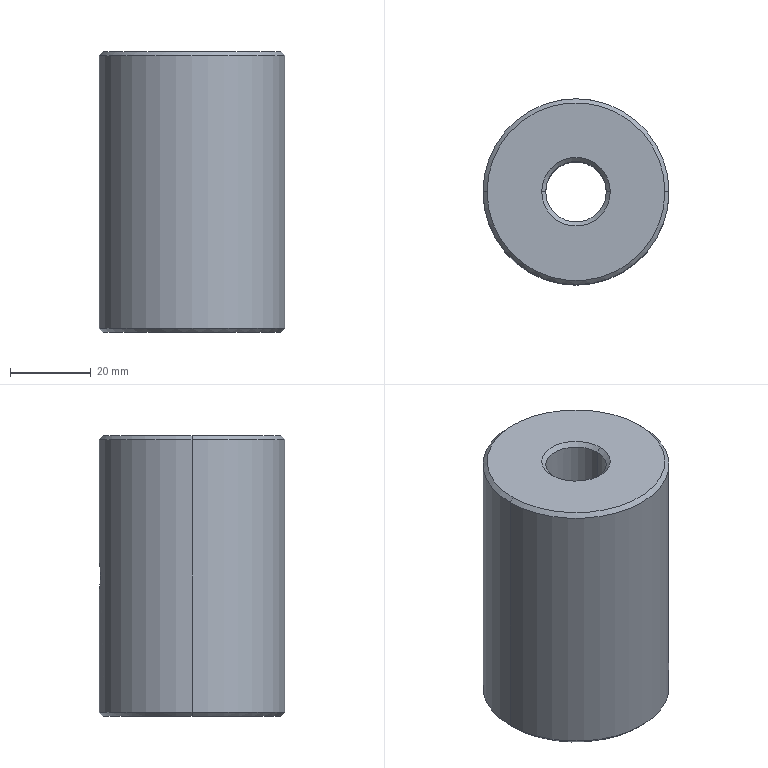Component | SolidWorks | Roller-01-2-1_XT-1-11-2-1 | 1 solid | 19 faces | box 46 x 46 x 69.5 mm | volume 102579 mm3 | cone 8 | cylinder 8 | plane 3 | commonest cylinder face diameters 4.5 x2 8 x2 15 x2 46 x2
STEP:
#1=CARTESIAN_POINT('',(17.806,2.81,-4.193));
#2=VERTEX_POINT('',#1);
#3=CARTESIAN_POINT('',(17.216,2.81,-4.193));
#4=VERTEX_POINT('',#3);
#5=CARTESIAN_POINT('',(17.511,2.81,-4.193));
#6=DIRECTION('',(0.,0.,-1.));
#7=DIRECTION('',(1.,0.,0.));
#8=AXIS2_PLACEMENT_3D('',#5,#6,#7);
#9=CIRCLE('',#8,0.2953);
#10=EDGE_CURVE('',#2,#4,#9,.T.);
#11=ORIENTED_EDGE('',*,*,#10,.F.);
#12=CARTESIAN_POINT('',(17.846,2.81,-4.232));
#13=VERTEX_POINT('',#12);
#14=CARTESIAN_POINT('',(17.846,2.81,-4.232));
#15=DIRECTION('',(0.7071,0.,-0.7071));
#16=VECTOR('',#15,39.37);
#17=LINE('',#14,#16);
#18=EDGE_CURVE('',#2,#13,#17,.T.);
#19=ORIENTED_EDGE('',*,*,#18,.T.);
#20=CARTESIAN_POINT('',(17.177,2.81,-4.232));
#21=VERTEX_POINT('',#20);
#22=CARTESIAN_POINT('',(17.511,2.81,-4.232));
#23=DIRECTION('',(0.,0.,1.));
#24=DIRECTION('',(1.,0.,0.));
#25=AXIS2_PLACEMENT_3D('',#22,#23,#24);
#26=CIRCLE('',#25,0.3346);
#27=EDGE_CURVE('',#21,#13,#26,.T.);
#28=ORIENTED_EDGE('',*,*,#27,.F.);
#29=CARTESIAN_POINT('',(17.177,2.81,-4.232));
#30=DIRECTION('',(-0.7071,0.,-0.7071));
#31=VECTOR('',#30,39.37);
#32=LINE('',#29,#31);
#33=EDGE_CURVE('',#4,#21,#32,.T.);
#34=ORIENTED_EDGE('',*,*,#33,.F.);
#35=EDGE_LOOP('',(#11,#19,#28,#34));
#36=FACE_OUTER_BOUND('',#35,.T.);
#37=CARTESIAN_POINT('',(17.511,2.81,-4.232));
#38=DIRECTION('',(0.,0.,-1.));
#39=DIRECTION('',(-1.,0.,0.));
#40=AXIS2_PLACEMENT_3D('',#37,#38,#39);
#41=CONICAL_SURFACE('',#40,0.3346,0.7854);
#42=ADVANCED_FACE('',(#36),#41,.F.);
#43=CARTESIAN_POINT('',(16.645,2.81,-4.232));
#44=VERTEX_POINT('',#43);
#45=CARTESIAN_POINT('',(18.377,2.81,-4.232));
#46=VERTEX_POINT('',#45);
#47=CARTESIAN_POINT('',(17.511,2.81,-4.232));
#48=DIRECTION('',(0.,0.,-1.));
#49=DIRECTION('',(1.,0.,0.));
#50=AXIS2_PLACEMENT_3D('',#47,#48,#49);
#51=CIRCLE('',#50,0.8661);
#52=EDGE_CURVE('',#44,#46,#51,.T.);
#53=ORIENTED_EDGE('',*,*,#52,.F.);
#54=CARTESIAN_POINT('',(16.606,2.81,-4.193));
#55=VERTEX_POINT('',#54);
#56=CARTESIAN_POINT('',(16.606,2.81,-4.193));
#57=DIRECTION('',(-0.7071,0.,0.7071));
#58=VECTOR('',#57,39.37);
#59=LINE('',#56,#58);
#60=EDGE_CURVE('',#44,#55,#59,.T.);
#61=ORIENTED_EDGE('',*,*,#60,.T.);
#62=CARTESIAN_POINT('',(18.417,2.81,-4.193));
#63=VERTEX_POINT('',#62);
#64=CARTESIAN_POINT('',(17.511,2.81,-4.193));
#65=DIRECTION('',(0.,0.,1.));
#66=DIRECTION('',(1.,0.,0.));
#67=AXIS2_PLACEMENT_3D('',#64,#65,#66);
#68=CIRCLE('',#67,0.9055);
#69=EDGE_CURVE('',#63,#55,#68,.T.);
#70=ORIENTED_EDGE('',*,*,#69,.F.);
#71=CARTESIAN_POINT('',(18.417,2.81,-4.193));
#72=DIRECTION('',(0.7071,0.,0.7071));
#73=VECTOR('',#72,39.37);
#74=LINE('',#71,#73);
#75=EDGE_CURVE('',#46,#63,#74,.T.);
#76=ORIENTED_EDGE('',*,*,#75,.F.);
#77=EDGE_LOOP('',(#53,#61,#70,#76));
#78=FACE_OUTER_BOUND('',#77,.T.);
#79=CARTESIAN_POINT('',(17.511,2.81,-4.193));
#80=DIRECTION('',(0.,0.,1.));
#81=DIRECTION('',(1.,0.,0.));
#82=AXIS2_PLACEMENT_3D('',#79,#80,#81);
#83=CONICAL_SURFACE('',#82,0.9055,0.7854);
#84=ADVANCED_FACE('',(#78),#83,.T.);
#85=CARTESIAN_POINT('',(18.377,2.81,-1.496));
#86=VERTEX_POINT('',#85);
#87=CARTESIAN_POINT('',(16.645,2.81,-1.496));
#88=VERTEX_POINT('',#87);
#89=CARTESIAN_POINT('',(17.511,2.81,-1.496));
#90=DIRECTION('',(0.,0.,1.));
#91=DIRECTION('',(1.,0.,0.));
#92=AXIS2_PLACEMENT_3D('',#89,#90,#91);
#93=CIRCLE('',#92,0.8661);
#94=EDGE_CURVE('',#86,#88,#93,.T.);
#95=ORIENTED_EDGE('',*,*,#94,.F.);
#96=CARTESIAN_POINT('',(18.417,2.81,-1.535));
#97=VERTEX_POINT('',#96);
#98=CARTESIAN_POINT('',(18.377,2.81,-1.496));
#99=DIRECTION('',(0.7071,0.,-0.7071));
#100=VECTOR('',#99,39.37);
#101=LINE('',#98,#100);
#102=EDGE_CURVE('',#86,#97,#101,.T.);
#103=ORIENTED_EDGE('',*,*,#102,.T.);
#104=CARTESIAN_POINT('',(16.606,2.81,-1.535));
#105=VERTEX_POINT('',#104);
#106=CARTESIAN_POINT('',(17.511,2.81,-1.535));
#107=DIRECTION('',(0.,0.,-1.));
#108=DIRECTION('',(1.,0.,0.));
#109=AXIS2_PLACEMENT_3D('',#106,#107,#108);
#110=CIRCLE('',#109,0.9055);
#111=EDGE_CURVE('',#105,#97,#110,.T.);
#112=ORIENTED_EDGE('',*,*,#111,.F.);
#113=CARTESIAN_POINT('',(16.645,2.81,-1.496));
#114=DIRECTION('',(-0.7071,0.,-0.7071));
#115=VECTOR('',#114,39.37);
#116=LINE('',#113,#115);
#117=EDGE_CURVE('',#88,#105,#116,.T.);
#118=ORIENTED_EDGE('',*,*,#117,.F.);
#119=EDGE_LOOP('',(#95,#103,#112,#118));
#120=FACE_OUTER_BOUND('',#119,.T.);
#121=CARTESIAN_POINT('',(17.511,2.81,-1.496));
#122=DIRECTION('',(0.,0.,-1.));
#123=DIRECTION('',(-1.,0.,0.));
#124=AXIS2_PLACEMENT_3D('',#121,#122,#123);
#125=CONICAL_SURFACE('',#124,0.8661,0.7854);
#126=ADVANCED_FACE('',(#120),#125,.T.);
#127=CARTESIAN_POINT('',(17.216,2.81,-1.535));
#128=VERTEX_POINT('',#127);
#129=CARTESIAN_POINT('',(17.806,2.81,-1.535));
#130=VERTEX_POINT('',#129);
#131=CARTESIAN_POINT('',(17.511,2.81,-1.535));
#132=DIRECTION('',(0.,0.,1.));
#133=DIRECTION('',(1.,0.,0.));
#134=AXIS2_PLACEMENT_3D('',#131,#132,#133);
#135=CIRCLE('',#134,0.2953);
#136=EDGE_CURVE('',#128,#130,#135,.T.);
#137=ORIENTED_EDGE('',*,*,#136,.F.);
#138=CARTESIAN_POINT('',(17.177,2.81,-1.496));
#139=VERTEX_POINT('',#138);
#140=CARTESIAN_POINT('',(17.216,2.81,-1.535));
#141=DIRECTION('',(-0.7071,0.,0.7071));
#142=VECTOR('',#141,39.37);
#143=LINE('',#140,#142);
#144=EDGE_CURVE('',#128,#139,#143,.T.);
#145=ORIENTED_EDGE('',*,*,#144,.T.);
#146=CARTESIAN_POINT('',(17.846,2.81,-1.496));
#147=VERTEX_POINT('',#146);
#148=CARTESIAN_POINT('',(17.511,2.81,-1.496));
#149=DIRECTION('',(0.,0.,-1.));
#150=DIRECTION('',(1.,0.,0.));
#151=AXIS2_PLACEMENT_3D('',#148,#149,#150);
#152=CIRCLE('',#151,0.3346);
#153=EDGE_CURVE('',#147,#139,#152,.T.);
#154=ORIENTED_EDGE('',*,*,#153,.F.);
#155=CARTESIAN_POINT('',(17.806,2.81,-1.535));
#156=DIRECTION('',(0.7071,0.,0.7071));
#157=VECTOR('',#156,39.37);
#158=LINE('',#155,#157);
#159=EDGE_CURVE('',#130,#147,#158,.T.);
#160=ORIENTED_EDGE('',*,*,#159,.F.);
#161=EDGE_LOOP('',(#137,#145,#154,#160));
#162=FACE_OUTER_BOUND('',#161,.T.);
#163=CARTESIAN_POINT('',(17.511,2.81,-1.535));
#164=DIRECTION('',(0.,0.,1.));
#165=DIRECTION('',(1.,0.,0.));
#166=AXIS2_PLACEMENT_3D('',#163,#164,#165);
#167=CONICAL_SURFACE('',#166,0.2953,0.7854);
#168=ADVANCED_FACE('',(#162),#167,.F.);
#169=CARTESIAN_POINT('',(17.511,3.106,-2.776));
#170=VERTEX_POINT('',#169);
#171=CARTESIAN_POINT('',(17.511,3.106,-2.953));
#172=VERTEX_POINT('',#171);
#173=CARTESIAN_POINT('',(17.511,3.106,-2.776));
#174=CARTESIAN_POINT('',(17.505,3.106,-2.776));
#175=CARTESIAN_POINT('',(17.499,3.106,-2.776));
#176=CARTESIAN_POINT('',(17.488,3.105,-2.778));
#177=CARTESIAN_POINT('',(17.482,3.104,-2.78));
#178=CARTESIAN_POINT('',(17.472,3.103,-2.785));
#179=CARTESIAN_POINT('',(17.467,3.102,-2.787));
#180=CARTESIAN_POINT('',(17.457,3.101,-2.794));
#181=CARTESIAN_POINT('',(17.453,3.1,-2.797));
#182=CARTESIAN_POINT('',(17.44,3.097,-2.81));
#183=CARTESIAN_POINT('',(17.434,3.095,-2.82));
#184=CARTESIAN_POINT('',(17.427,3.094,-2.835));
#185=CARTESIAN_POINT('',(17.425,3.093,-2.841));
#186=CARTESIAN_POINT('',(17.423,3.092,-2.853));
#187=CARTESIAN_POINT('',(17.423,3.092,-2.858));
#188=CARTESIAN_POINT('',(17.423,3.092,-2.87));
#189=CARTESIAN_POINT('',(17.423,3.092,-2.876));
#190=CARTESIAN_POINT('',(17.425,3.093,-2.887));
#191=CARTESIAN_POINT('',(17.427,3.094,-2.893));
#192=CARTESIAN_POINT('',(17.434,3.095,-2.909));
#193=CARTESIAN_POINT('',(17.44,3.097,-2.919));
#194=CARTESIAN_POINT('',(17.453,3.1,-2.931));
#195=CARTESIAN_POINT('',(17.457,3.101,-2.935));
#196=CARTESIAN_POINT('',(17.467,3.102,-2.941));
#197=CARTESIAN_POINT('',(17.472,3.103,-2.944));
#198=CARTESIAN_POINT('',(17.483,3.104,-2.948));
#199=CARTESIAN_POINT('',(17.488,3.105,-2.95));
#200=CARTESIAN_POINT('',(17.499,3.106,-2.952));
#201=CARTESIAN_POINT('',(17.505,3.106,-2.953));
#202=CARTESIAN_POINT('',(17.511,3.106,-2.953));
#203=B_SPLINE_CURVE_WITH_KNOTS('',3,(#173,#174,#175,#176,#177,#178,#179,#180,#181,#182,#183,#184,#185,#186,#187,#188,#189,#190,#191,#192,#193,#194,#195,#196,#197,#198,#199,#200,#201,#202),.UNSPECIFIED.,.F.,.F.,(4,2,2,2,2,2,2,2,2,2,2,2,2,2,4),(0.,0.0004422,0.0008844,0.001327,0.001769,0.002653,0.003096,0.003538,0.00398,0.004422,0.005307,0.005749,0.006191,0.006633,0.007076),.UNSPECIFIED.);
#204=EDGE_CURVE('',#170,#172,#203,.T.);
#205=ORIENTED_EDGE('',*,*,#204,.T.);
#206=CARTESIAN_POINT('',(17.511,3.48,-2.953));
#207=VERTEX_POINT('',#206);
#208=CARTESIAN_POINT('',(17.511,3.716,-2.953));
#209=DIRECTION('',(0.,1.,0.));
#210=VECTOR('',#209,39.37);
#211=LINE('',#208,#210);
#212=EDGE_CURVE('',#172,#207,#211,.T.);
#213=ORIENTED_EDGE('',*,*,#212,.T.);
#214=CARTESIAN_POINT('',(17.511,3.48,-2.776));
#215=VERTEX_POINT('',#214);
#216=CARTESIAN_POINT('',(17.511,3.48,-2.864));
#217=DIRECTION('',(0.,1.,0.));
#218=DIRECTION('',(0.,0.,1.));
#219=AXIS2_PLACEMENT_3D('',#216,#217,#218);
#220=CIRCLE('',#219,0.08858);
#221=EDGE_CURVE('',#207,#215,#220,.T.);
#222=ORIENTED_EDGE('',*,*,#221,.T.);
#223=CARTESIAN_POINT('',(17.511,3.716,-2.776));
#224=DIRECTION('',(0.,1.,0.));
#225=VECTOR('',#224,39.37);
#226=LINE('',#223,#225);
#227=EDGE_CURVE('',#170,#215,#226,.T.);
#228=ORIENTED_EDGE('',*,*,#227,.F.);
#229=EDGE_LOOP('',(#205,#213,#222,#228));
#230=FACE_OUTER_BOUND('',#229,.T.);
#231=CARTESIAN_POINT('',(17.511,3.716,-2.864));
#232=DIRECTION('',(0.,1.,0.));
#233=DIRECTION('',(0.,0.,1.));
#234=AXIS2_PLACEMENT_3D('',#231,#232,#233);
#235=CYLINDRICAL_SURFACE('',#234,0.08858);
#236=ADVANCED_FACE('',(#230),#235,.F.);
#237=CARTESIAN_POINT('',(17.511,3.48,-3.022));
#238=VERTEX_POINT('',#237);
#239=CARTESIAN_POINT('',(17.511,3.48,-2.707));
#240=VERTEX_POINT('',#239);
#241=CARTESIAN_POINT('',(17.511,3.48,-2.864));
#242=DIRECTION('',(0.,1.,0.));
#243=DIRECTION('',(0.,0.,1.));
#244=AXIS2_PLACEMENT_3D('',#241,#242,#243);
#245=CIRCLE('',#244,0.1575);
#246=EDGE_CURVE('',#238,#240,#245,.T.);
#247=ORIENTED_EDGE('',*,*,#246,.F.);
#248=CARTESIAN_POINT('',(17.511,3.716,-3.022));
#249=VERTEX_POINT('',#248);
#250=CARTESIAN_POINT('',(17.511,3.716,-3.022));
#251=DIRECTION('',(0.,1.,0.));
#252=VECTOR('',#251,39.37);
#253=LINE('',#250,#252);
#254=EDGE_CURVE('',#238,#249,#253,.T.);
#255=ORIENTED_EDGE('',*,*,#254,.T.);
#256=CARTESIAN_POINT('',(17.511,3.716,-2.707));
#257=VERTEX_POINT('',#256);
#258=CARTESIAN_POINT('',(17.511,3.716,-2.707));
#259=CARTESIAN_POINT('',(17.501,3.716,-2.707));
#260=CARTESIAN_POINT('',(17.49,3.716,-2.708));
#261=CARTESIAN_POINT('',(17.47,3.715,-2.712));
#262=CARTESIAN_POINT('',(17.46,3.715,-2.715));
#263=CARTESIAN_POINT('',(17.441,3.713,-2.723));
#264=CARTESIAN_POINT('',(17.432,3.713,-2.728));
#265=CARTESIAN_POINT('',(17.415,3.711,-2.739));
#266=CARTESIAN_POINT('',(17.407,3.71,-2.746));
#267=CARTESIAN_POINT('',(17.393,3.708,-2.76));
#268=CARTESIAN_POINT('',(17.386,3.707,-2.768));
#269=CARTESIAN_POINT('',(17.375,3.706,-2.785));
#270=CARTESIAN_POINT('',(17.37,3.705,-2.794));
#271=CARTESIAN_POINT('',(17.362,3.704,-2.813));
#272=CARTESIAN_POINT('',(17.359,3.703,-2.823));
#273=CARTESIAN_POINT('',(17.355,3.702,-2.844));
#274=CARTESIAN_POINT('',(17.354,3.702,-2.854));
#275=CARTESIAN_POINT('',(17.354,3.702,-2.874));
#276=CARTESIAN_POINT('',(17.355,3.702,-2.885));
#277=CARTESIAN_POINT('',(17.359,3.703,-2.905));
#278=CARTESIAN_POINT('',(17.362,3.704,-2.915));
#279=CARTESIAN_POINT('',(17.37,3.705,-2.934));
#280=CARTESIAN_POINT('',(17.375,3.706,-2.943));
#281=CARTESIAN_POINT('',(17.386,3.707,-2.96));
#282=CARTESIAN_POINT('',(17.392,3.708,-2.968));
#283=CARTESIAN_POINT('',(17.407,3.71,-2.983));
#284=CARTESIAN_POINT('',(17.415,3.711,-2.989));
#285=CARTESIAN_POINT('',(17.432,3.713,-3.001));
#286=CARTESIAN_POINT('',(17.441,3.713,-3.006));
#287=CARTESIAN_POINT('',(17.46,3.715,-3.014));
#288=CARTESIAN_POINT('',(17.47,3.715,-3.017));
#289=CARTESIAN_POINT('',(17.49,3.716,-3.021));
#290=CARTESIAN_POINT('',(17.501,3.716,-3.022));
#291=CARTESIAN_POINT('',(17.511,3.716,-3.022));
#292=B_SPLINE_CURVE_WITH_KNOTS('',3,(#258,#259,#260,#261,#262,#263,#264,#265,#266,#267,#268,#269,#270,#271,#272,#273,#274,#275,#276,#277,#278,#279,#280,#281,#282,#283,#284,#285,#286,#287,#288,#289,#290,#291),.UNSPECIFIED.,.F.,.F.,(4,2,2,2,2,2,2,2,2,2,2,2,2,2,2,2,4),(0.,0.0007831,0.001566,0.002349,0.003132,0.003916,0.004699,0.005482,0.006265,0.007048,0.007831,0.008614,0.009397,0.01018,0.01096,0.01175,0.01253),.UNSPECIFIED.);
#293=EDGE_CURVE('',#257,#249,#292,.T.);
#294=ORIENTED_EDGE('',*,*,#293,.F.);
#295=CARTESIAN_POINT('',(17.511,3.716,-2.707));
#296=DIRECTION('',(0.,1.,0.));
#297=VECTOR('',#296,39.37);
#298=LINE('',#295,#297);
#299=EDGE_CURVE('',#240,#257,#298,.T.);
#300=ORIENTED_EDGE('',*,*,#299,.F.);
#301=EDGE_LOOP('',(#247,#255,#294,#300));
#302=FACE_OUTER_BOUND('',#301,.T.);
#303=CARTESIAN_POINT('',(17.511,3.716,-2.864));
#304=DIRECTION('',(0.,1.,0.));
#305=DIRECTION('',(0.,0.,1.));
#306=AXIS2_PLACEMENT_3D('',#303,#304,#305);
#307=CYLINDRICAL_SURFACE('',#306,0.1575);
#308=ADVANCED_FACE('',(#302),#307,.F.);
#309=ORIENTED_EDGE('',*,*,#136,.T.);
#310=CARTESIAN_POINT('',(17.806,2.81,-1.496));
#311=DIRECTION('',(0.,0.,-1.));
#312=VECTOR('',#311,39.37);
#313=LINE('',#310,#312);
#314=EDGE_CURVE('',#130,#2,#313,.T.);
#315=ORIENTED_EDGE('',*,*,#314,.T.);
#316=ORIENTED_EDGE('',*,*,#10,.T.);
#317=CARTESIAN_POINT('',(17.216,2.81,-1.496));
#318=DIRECTION('',(0.,0.,-1.));
#319=VECTOR('',#318,39.37);
#320=LINE('',#317,#319);
#321=EDGE_CURVE('',#128,#4,#320,.T.);
#322=ORIENTED_EDGE('',*,*,#321,.F.);
#323=EDGE_LOOP('',(#309,#315,#316,#322));
#324=FACE_OUTER_BOUND('',#323,.T.);
#325=CARTESIAN_POINT('',(17.511,2.81,-1.496));
#326=DIRECTION('',(0.,0.,-1.));
#327=DIRECTION('',(-1.,0.,0.));
#328=AXIS2_PLACEMENT_3D('',#325,#326,#327);
#329=CYLINDRICAL_SURFACE('',#328,0.2953);
#330=ADVANCED_FACE('',(#324),#329,.F.);
#331=ORIENTED_EDGE('',*,*,#293,.T.);
#332=CARTESIAN_POINT('',(17.511,3.716,-3.022));
#333=CARTESIAN_POINT('',(17.521,3.716,-3.022));
#334=CARTESIAN_POINT('',(17.532,3.716,-3.021));
#335=CARTESIAN_POINT('',(17.552,3.715,-3.017));
#336=CARTESIAN_POINT('',(17.562,3.715,-3.014));
#337=CARTESIAN_POINT('',(17.581,3.713,-3.006));
#338=CARTESIAN_POINT('',(17.59,3.713,-3.001));
#339=CARTESIAN_POINT('',(17.607,3.711,-2.989));
#340=CARTESIAN_POINT('',(17.615,3.71,-2.983));
#341=CARTESIAN_POINT('',(17.63,3.708,-2.968));
#342=CARTESIAN_POINT('',(17.636,3.707,-2.96));
#343=CARTESIAN_POINT('',(17.648,3.706,-2.943));
#344=CARTESIAN_POINT('',(17.653,3.705,-2.934));
#345=CARTESIAN_POINT('',(17.661,3.704,-2.915));
#346=CARTESIAN_POINT('',(17.664,3.703,-2.905));
#347=CARTESIAN_POINT('',(17.668,3.702,-2.885));
#348=CARTESIAN_POINT('',(17.669,3.702,-2.875));
#349=CARTESIAN_POINT('',(17.669,3.702,-2.854));
#350=CARTESIAN_POINT('',(17.668,3.702,-2.844));
#351=CARTESIAN_POINT('',(17.664,3.703,-2.823));
#352=CARTESIAN_POINT('',(17.661,3.704,-2.813));
#353=CARTESIAN_POINT('',(17.653,3.705,-2.794));
#354=CARTESIAN_POINT('',(17.648,3.706,-2.785));
#355=CARTESIAN_POINT('',(17.636,3.707,-2.768));
#356=CARTESIAN_POINT('',(17.63,3.708,-2.76));
#357=CARTESIAN_POINT('',(17.615,3.71,-2.746));
#358=CARTESIAN_POINT('',(17.607,3.711,-2.739));
#359=CARTESIAN_POINT('',(17.59,3.713,-2.728));
#360=CARTESIAN_POINT('',(17.581,3.713,-2.723));
#361=CARTESIAN_POINT('',(17.562,3.715,-2.715));
#362=CARTESIAN_POINT('',(17.552,3.715,-2.712));
#363=CARTESIAN_POINT('',(17.532,3.716,-2.708));
#364=CARTESIAN_POINT('',(17.522,3.716,-2.707));
#365=CARTESIAN_POINT('',(17.511,3.716,-2.707));
#366=B_SPLINE_CURVE_WITH_KNOTS('',3,(#332,#333,#334,#335,#336,#337,#338,#339,#340,#341,#342,#343,#344,#345,#346,#347,#348,#349,#350,#351,#352,#353,#354,#355,#356,#357,#358,#359,#360,#361,#362,#363,#364,#365),.UNSPECIFIED.,.F.,.F.,(4,2,2,2,2,2,2,2,2,2,2,2,2,2,2,2,4),(0.01253,0.01331,0.0141,0.01488,0.01566,0.01644,0.01723,0.01801,0.01879,0.01958,0.02036,0.02114,0.02192,0.02271,0.02349,0.02427,0.02506),.UNSPECIFIED.);
#367=EDGE_CURVE('',#249,#257,#366,.T.);
#368=ORIENTED_EDGE('',*,*,#367,.T.);
#369=EDGE_LOOP('',(#331,#368));
#370=FACE_BOUND('',#369,.T.);
#371=ORIENTED_EDGE('',*,*,#111,.T.);
#372=CARTESIAN_POINT('',(18.417,2.81,-1.496));
#373=DIRECTION('',(0.,0.,-1.));
#374=VECTOR('',#373,39.37);
#375=LINE('',#372,#374);
#376=EDGE_CURVE('',#97,#63,#375,.T.);
#377=ORIENTED_EDGE('',*,*,#376,.T.);
#378=ORIENTED_EDGE('',*,*,#69,.T.);
#379=CARTESIAN_POINT('',(16.606,2.81,-1.496));
#380=DIRECTION('',(0.,0.,-1.));
#381=VECTOR('',#380,39.37);
#382=LINE('',#379,#381);
#383=EDGE_CURVE('',#105,#55,#382,.T.);
#384=ORIENTED_EDGE('',*,*,#383,.F.);
#385=EDGE_LOOP('',(#371,#377,#378,#384));
#386=FACE_OUTER_BOUND('',#385,.T.);
#387=CARTESIAN_POINT('',(17.511,2.81,-1.496));
#388=DIRECTION('',(0.,0.,-1.));
#389=DIRECTION('',(-1.,0.,0.));
#390=AXIS2_PLACEMENT_3D('',#387,#388,#389);
#391=CYLINDRICAL_SURFACE('',#390,0.9055);
#392=ADVANCED_FACE('',(#370,#386),#391,.T.);
#393=ORIENTED_EDGE('',*,*,#153,.T.);
#394=CARTESIAN_POINT('',(17.511,2.81,-1.496));
#395=DIRECTION('',(0.,0.,-1.));
#396=DIRECTION('',(1.,0.,0.));
#397=AXIS2_PLACEMENT_3D('',#394,#395,#396);
#398=CIRCLE('',#397,0.3346);
#399=EDGE_CURVE('',#139,#147,#398,.T.);
#400=ORIENTED_EDGE('',*,*,#399,.T.);
#401=EDGE_LOOP('',(#393,#400));
#402=FACE_BOUND('',#401,.T.);
#403=CARTESIAN_POINT('',(17.511,2.81,-1.496));
#404=DIRECTION('',(0.,0.,1.));
#405=DIRECTION('',(1.,0.,0.));
#406=AXIS2_PLACEMENT_3D('',#403,#404,#405);
#407=CIRCLE('',#406,0.8661);
#408=EDGE_CURVE('',#88,#86,#407,.T.);
#409=ORIENTED_EDGE('',*,*,#408,.T.);
#410=ORIENTED_EDGE('',*,*,#94,.T.);
#411=EDGE_LOOP('',(#409,#410));
#412=FACE_OUTER_BOUND('',#411,.T.);
#413=CARTESIAN_POINT('',(17.511,2.81,-1.496));
#414=DIRECTION('',(0.,0.,1.));
#415=DIRECTION('',(1.,0.,0.));
#416=AXIS2_PLACEMENT_3D('',#413,#414,#415);
#417=PLANE('',#416);
#418=ADVANCED_FACE('',(#402,#412),#417,.T.);
#419=CARTESIAN_POINT('',(17.511,2.81,-4.232));
#420=DIRECTION('',(0.,0.,-1.));
#421=DIRECTION('',(1.,0.,0.));
#422=AXIS2_PLACEMENT_3D('',#419,#420,#421);
#423=CIRCLE('',#422,0.8661);
#424=EDGE_CURVE('',#46,#44,#423,.T.);
#425=ORIENTED_EDGE('',*,*,#424,.T.);
#426=ORIENTED_EDGE('',*,*,#52,.T.);
#427=EDGE_LOOP('',(#425,#426));
#428=FACE_OUTER_BOUND('',#427,.T.);
#429=ORIENTED_EDGE('',*,*,#27,.T.);
#430=CARTESIAN_POINT('',(17.511,2.81,-4.232));
#431=DIRECTION('',(0.,0.,1.));
#432=DIRECTION('',(1.,0.,0.));
#433=AXIS2_PLACEMENT_3D('',#430,#431,#432);
#434=CIRCLE('',#433,0.3346);
#435=EDGE_CURVE('',#13,#21,#434,.T.);
#436=ORIENTED_EDGE('',*,*,#435,.T.);
#437=EDGE_LOOP('',(#429,#436));
#438=FACE_BOUND('',#437,.T.);
#439=CARTESIAN_POINT('',(17.511,2.81,-4.232));
#440=DIRECTION('',(0.,0.,1.));
#441=DIRECTION('',(1.,0.,0.));
#442=AXIS2_PLACEMENT_3D('',#439,#440,#441);
#443=PLANE('',#442);
#444=ADVANCED_FACE('',(#428,#438),#443,.F.);
#445=ORIENTED_EDGE('',*,*,#376,.F.);
#446=CARTESIAN_POINT('',(17.511,2.81,-1.535));
#447=DIRECTION('',(0.,0.,-1.));
#448=DIRECTION('',(1.,0.,0.));
#449=AXIS2_PLACEMENT_3D('',#446,#447,#448);
#450=CIRCLE('',#449,0.9055);
#451=EDGE_CURVE('',#97,#105,#450,.T.);
#452=ORIENTED_EDGE('',*,*,#451,.T.);
#453=ORIENTED_EDGE('',*,*,#383,.T.);
#454=CARTESIAN_POINT('',(17.511,2.81,-4.193));
#455=DIRECTION('',(0.,0.,1.));
#456=DIRECTION('',(1.,0.,0.));
#457=AXIS2_PLACEMENT_3D('',#454,#455,#456);
#458=CIRCLE('',#457,0.9055);
#459=EDGE_CURVE('',#55,#63,#458,.T.);
#460=ORIENTED_EDGE('',*,*,#459,.T.);
#461=EDGE_LOOP('',(#445,#452,#453,#460));
#462=FACE_OUTER_BOUND('',#461,.T.);
#463=CARTESIAN_POINT('',(17.511,2.81,-1.496));
#464=DIRECTION('',(0.,0.,-1.));
#465=DIRECTION('',(-1.,0.,0.));
#466=AXIS2_PLACEMENT_3D('',#463,#464,#465);
#467=CYLINDRICAL_SURFACE('',#466,0.9055);
#468=ADVANCED_FACE('',(#462),#467,.T.);
#469=ORIENTED_EDGE('',*,*,#314,.F.);
#470=CARTESIAN_POINT('',(17.511,2.81,-1.535));
#471=DIRECTION('',(0.,0.,1.));
#472=DIRECTION('',(1.,0.,0.));
#473=AXIS2_PLACEMENT_3D('',#470,#471,#472);
#474=CIRCLE('',#473,0.2953);
#475=EDGE_CURVE('',#130,#128,#474,.T.);
#476=ORIENTED_EDGE('',*,*,#475,.T.);
#477=ORIENTED_EDGE('',*,*,#321,.T.);
#478=CARTESIAN_POINT('',(17.511,2.81,-4.193));
#479=DIRECTION('',(0.,0.,-1.));
#480=DIRECTION('',(1.,0.,0.));
#481=AXIS2_PLACEMENT_3D('',#478,#479,#480);
#482=CIRCLE('',#481,0.2953);
#483=EDGE_CURVE('',#4,#2,#482,.T.);
#484=ORIENTED_EDGE('',*,*,#483,.T.);
#485=EDGE_LOOP('',(#469,#476,#477,#484));
#486=FACE_OUTER_BOUND('',#485,.T.);
#487=ORIENTED_EDGE('',*,*,#204,.F.);
#488=CARTESIAN_POINT('',(17.511,3.106,-2.953));
#489=CARTESIAN_POINT('',(17.523,3.106,-2.953));
#490=CARTESIAN_POINT('',(17.534,3.105,-2.95));
#491=CARTESIAN_POINT('',(17.55,3.103,-2.944));
#492=CARTESIAN_POINT('',(17.556,3.102,-2.941));
#493=CARTESIAN_POINT('',(17.565,3.101,-2.935));
#494=CARTESIAN_POINT('',(17.57,3.1,-2.931));
#495=CARTESIAN_POINT('',(17.578,3.098,-2.923));
#496=CARTESIAN_POINT('',(17.582,3.097,-2.918));
#497=CARTESIAN_POINT('',(17.588,3.096,-2.909));
#498=CARTESIAN_POINT('',(17.591,3.095,-2.904));
#499=CARTESIAN_POINT('',(17.595,3.094,-2.893));
#500=CARTESIAN_POINT('',(17.597,3.093,-2.887));
#501=CARTESIAN_POINT('',(17.599,3.092,-2.876));
#502=CARTESIAN_POINT('',(17.6,3.092,-2.87));
#503=CARTESIAN_POINT('',(17.6,3.092,-2.858));
#504=CARTESIAN_POINT('',(17.599,3.092,-2.853));
#505=CARTESIAN_POINT('',(17.597,3.093,-2.841));
#506=CARTESIAN_POINT('',(17.595,3.094,-2.836));
#507=CARTESIAN_POINT('',(17.589,3.095,-2.82));
#508=CARTESIAN_POINT('',(17.582,3.097,-2.81));
#509=CARTESIAN_POINT('',(17.57,3.1,-2.797));
#510=CARTESIAN_POINT('',(17.565,3.101,-2.794));
#511=CARTESIAN_POINT('',(17.556,3.102,-2.787));
#512=CARTESIAN_POINT('',(17.551,3.103,-2.785));
#513=CARTESIAN_POINT('',(17.54,3.104,-2.78));
#514=CARTESIAN_POINT('',(17.534,3.105,-2.778));
#515=CARTESIAN_POINT('',(17.523,3.106,-2.776));
#516=CARTESIAN_POINT('',(17.517,3.106,-2.776));
#517=CARTESIAN_POINT('',(17.511,3.106,-2.776));
#518=B_SPLINE_CURVE_WITH_KNOTS('',3,(#488,#489,#490,#491,#492,#493,#494,#495,#496,#497,#498,#499,#500,#501,#502,#503,#504,#505,#506,#507,#508,#509,#510,#511,#512,#513,#514,#515,#516,#517),.UNSPECIFIED.,.F.,.F.,(4,2,2,2,2,2,2,2,2,2,2,2,2,2,4),(0.007076,0.00796,0.008402,0.008844,0.009286,0.009728,0.01017,0.01061,0.01105,0.0115,0.01238,0.01282,0.01326,0.01371,0.01415),.UNSPECIFIED.);
#519=EDGE_CURVE('',#172,#170,#518,.T.);
#520=ORIENTED_EDGE('',*,*,#519,.F.);
#521=EDGE_LOOP('',(#487,#520));
#522=FACE_BOUND('',#521,.T.);
#523=CARTESIAN_POINT('',(17.511,2.81,-1.496));
#524=DIRECTION('',(0.,0.,-1.));
#525=DIRECTION('',(-1.,0.,0.));
#526=AXIS2_PLACEMENT_3D('',#523,#524,#525);
#527=CYLINDRICAL_SURFACE('',#526,0.2953);
#528=ADVANCED_FACE('',(#486,#522),#527,.F.);
#529=ORIENTED_EDGE('',*,*,#254,.F.);
#530=CARTESIAN_POINT('',(17.511,3.48,-2.864));
#531=DIRECTION('',(0.,1.,0.));
#532=DIRECTION('',(0.,0.,1.));
#533=AXIS2_PLACEMENT_3D('',#530,#531,#532);
#534=CIRCLE('',#533,0.1575);
#535=EDGE_CURVE('',#240,#238,#534,.T.);
#536=ORIENTED_EDGE('',*,*,#535,.F.);
#537=ORIENTED_EDGE('',*,*,#299,.T.);
#538=ORIENTED_EDGE('',*,*,#367,.F.);
#539=EDGE_LOOP('',(#529,#536,#537,#538));
#540=FACE_OUTER_BOUND('',#539,.T.);
#541=CARTESIAN_POINT('',(17.511,3.716,-2.864));
#542=DIRECTION('',(0.,1.,0.));
#543=DIRECTION('',(0.,0.,1.));
#544=AXIS2_PLACEMENT_3D('',#541,#542,#543);
#545=CYLINDRICAL_SURFACE('',#544,0.1575);
#546=ADVANCED_FACE('',(#540),#545,.F.);
#547=ORIENTED_EDGE('',*,*,#212,.F.);
#548=ORIENTED_EDGE('',*,*,#519,.T.);
#549=ORIENTED_EDGE('',*,*,#227,.T.);
#550=CARTESIAN_POINT('',(17.511,3.48,-2.864));
#551=DIRECTION('',(0.,1.,0.));
#552=DIRECTION('',(0.,0.,1.));
#553=AXIS2_PLACEMENT_3D('',#550,#551,#552);
#554=CIRCLE('',#553,0.08858);
#555=EDGE_CURVE('',#215,#207,#554,.T.);
#556=ORIENTED_EDGE('',*,*,#555,.T.);
#557=EDGE_LOOP('',(#547,#548,#549,#556));
#558=FACE_OUTER_BOUND('',#557,.T.);
#559=CARTESIAN_POINT('',(17.511,3.716,-2.864));
#560=DIRECTION('',(0.,1.,0.));
#561=DIRECTION('',(0.,0.,1.));
#562=AXIS2_PLACEMENT_3D('',#559,#560,#561);
#563=CYLINDRICAL_SURFACE('',#562,0.08858);
#564=ADVANCED_FACE('',(#558),#563,.F.);
#565=ORIENTED_EDGE('',*,*,#555,.F.);
#566=ORIENTED_EDGE('',*,*,#221,.F.);
#567=EDGE_LOOP('',(#565,#566));
#568=FACE_BOUND('',#567,.T.);
#569=ORIENTED_EDGE('',*,*,#535,.T.);
#570=ORIENTED_EDGE('',*,*,#246,.T.);
#571=EDGE_LOOP('',(#569,#570));
#572=FACE_OUTER_BOUND('',#571,.T.);
#573=CARTESIAN_POINT('',(17.6,3.48,-2.864));
#574=DIRECTION('',(0.,-1.,0.));
#575=DIRECTION('',(0.,0.,-1.));
#576=AXIS2_PLACEMENT_3D('',#573,#574,#575);
#577=PLANE('',#576);
#578=ADVANCED_FACE('',(#568,#572),#577,.F.);
#579=ORIENTED_EDGE('',*,*,#144,.F.);
#580=ORIENTED_EDGE('',*,*,#475,.F.);
#581=ORIENTED_EDGE('',*,*,#159,.T.);
#582=ORIENTED_EDGE('',*,*,#399,.F.);
#583=EDGE_LOOP('',(#579,#580,#581,#582));
#584=FACE_OUTER_BOUND('',#583,.T.);
#585=CARTESIAN_POINT('',(17.511,2.81,-1.535));
#586=DIRECTION('',(0.,0.,1.));
#587=DIRECTION('',(1.,0.,0.));
#588=AXIS2_PLACEMENT_3D('',#585,#586,#587);
#589=CONICAL_SURFACE('',#588,0.2953,0.7854);
#590=ADVANCED_FACE('',(#584),#589,.F.);
#591=ORIENTED_EDGE('',*,*,#102,.F.);
#592=ORIENTED_EDGE('',*,*,#408,.F.);
#593=ORIENTED_EDGE('',*,*,#117,.T.);
#594=ORIENTED_EDGE('',*,*,#451,.F.);
#595=EDGE_LOOP('',(#591,#592,#593,#594));
#596=FACE_OUTER_BOUND('',#595,.T.);
#597=CARTESIAN_POINT('',(17.511,2.81,-1.496));
#598=DIRECTION('',(0.,0.,-1.));
#599=DIRECTION('',(-1.,0.,0.));
#600=AXIS2_PLACEMENT_3D('',#597,#598,#599);
#601=CONICAL_SURFACE('',#600,0.8661,0.7854);
#602=ADVANCED_FACE('',(#596),#601,.T.);
#603=ORIENTED_EDGE('',*,*,#60,.F.);
#604=ORIENTED_EDGE('',*,*,#424,.F.);
#605=ORIENTED_EDGE('',*,*,#75,.T.);
#606=ORIENTED_EDGE('',*,*,#459,.F.);
#607=EDGE_LOOP('',(#603,#604,#605,#606));
#608=FACE_OUTER_BOUND('',#607,.T.);
#609=CARTESIAN_POINT('',(17.511,2.81,-4.193));
#610=DIRECTION('',(0.,0.,1.));
#611=DIRECTION('',(1.,0.,0.));
#612=AXIS2_PLACEMENT_3D('',#609,#610,#611);
#613=CONICAL_SURFACE('',#612,0.9055,0.7854);
#614=ADVANCED_FACE('',(#608),#613,.T.);
#615=ORIENTED_EDGE('',*,*,#18,.F.);
#616=ORIENTED_EDGE('',*,*,#483,.F.);
#617=ORIENTED_EDGE('',*,*,#33,.T.);
#618=ORIENTED_EDGE('',*,*,#435,.F.);
#619=EDGE_LOOP('',(#615,#616,#617,#618));
#620=FACE_OUTER_BOUND('',#619,.T.);
#621=CARTESIAN_POINT('',(17.511,2.81,-4.232));
#622=DIRECTION('',(0.,0.,-1.));
#623=DIRECTION('',(-1.,0.,0.));
#624=AXIS2_PLACEMENT_3D('',#621,#622,#623);
#625=CONICAL_SURFACE('',#624,0.3346,0.7854);
#626=ADVANCED_FACE('',(#620),#625,.F.);
#627=CLOSED_SHELL('',(#42,#84,#126,#168,#236,#308,#330,#392,#418,#444,#468,#528,#546,#564,#578,#590,#602,#614,#626));
#628=MANIFOLD_SOLID_BREP('',#627);
#629=CARTESIAN_POINT('',(0.,0.,0.));
#630=DIRECTION('',(0.,0.,1.));
#631=DIRECTION('',(1.,0.,0.));
#632=AXIS2_PLACEMENT_3D('',#629,#630,#631);
#633=(LENGTH_UNIT()NAMED_UNIT(*)SI_UNIT($,.METRE.));
#634=LENGTH_MEASURE_WITH_UNIT(LENGTH_MEASURE(0.0254),#633);
#635=DIMENSIONAL_EXPONENTS(1.,0.,0.,0.,0.,0.,0.);
#636=(CONVERSION_BASED_UNIT('',#634)LENGTH_UNIT()NAMED_UNIT(#635));
#637=UNCERTAINTY_MEASURE_WITH_UNIT(LENGTH_MEASURE(0.00001),#636,'','');
#638=(NAMED_UNIT(*)PLANE_ANGLE_UNIT()SI_UNIT($,.RADIAN.));
#639=(NAMED_UNIT(*)SI_UNIT($,.STERADIAN.)SOLID_ANGLE_UNIT());
#640=(GEOMETRIC_REPRESENTATION_CONTEXT(3)GLOBAL_UNCERTAINTY_ASSIGNED_CONTEXT((#637))GLOBAL_UNIT_ASSIGNED_CONTEXT((#636,#638,#639))REPRESENTATION_CONTEXT('',''));
#641=ADVANCED_BREP_SHAPE_REPRESENTATION('',(#628,#632),#640);
#642=COLOUR_RGB('',0.7922,0.8196,0.9333);
#643=FILL_AREA_STYLE_COLOUR('',#642);
#644=FILL_AREA_STYLE('',(#643));
#645=SURFACE_STYLE_FILL_AREA(#644);
#646=SURFACE_SIDE_STYLE('',(#645));
#647=SURFACE_STYLE_USAGE(.BOTH.,#646);
#648=PRESENTATION_STYLE_ASSIGNMENT((#647));
#649=STYLED_ITEM('',(#648),#628);
#650=(LENGTH_UNIT()NAMED_UNIT(*)SI_UNIT($,.METRE.));
#651=LENGTH_MEASURE_WITH_UNIT(LENGTH_MEASURE(0.0254),#650);
#652=DIMENSIONAL_EXPONENTS(1.,0.,0.,0.,0.,0.,0.);
#653=(CONVERSION_BASED_UNIT('',#651)LENGTH_UNIT()NAMED_UNIT(#652));
#654=UNCERTAINTY_MEASURE_WITH_UNIT(LENGTH_MEASURE(0.00001),#653,'','');
#655=(NAMED_UNIT(*)PLANE_ANGLE_UNIT()SI_UNIT($,.RADIAN.));
#656=(NAMED_UNIT(*)SI_UNIT($,.STERADIAN.)SOLID_ANGLE_UNIT());
#657=(GEOMETRIC_REPRESENTATION_CONTEXT(3)GLOBAL_UNCERTAINTY_ASSIGNED_CONTEXT((#654))GLOBAL_UNIT_ASSIGNED_CONTEXT((#653,#655,#656))REPRESENTATION_CONTEXT('',''));
#658=MECHANICAL_DESIGN_GEOMETRIC_PRESENTATION_REPRESENTATION('',(#649),#657);
#659=PRESENTATION_LAYER_ASSIGNMENT('','',(#649));